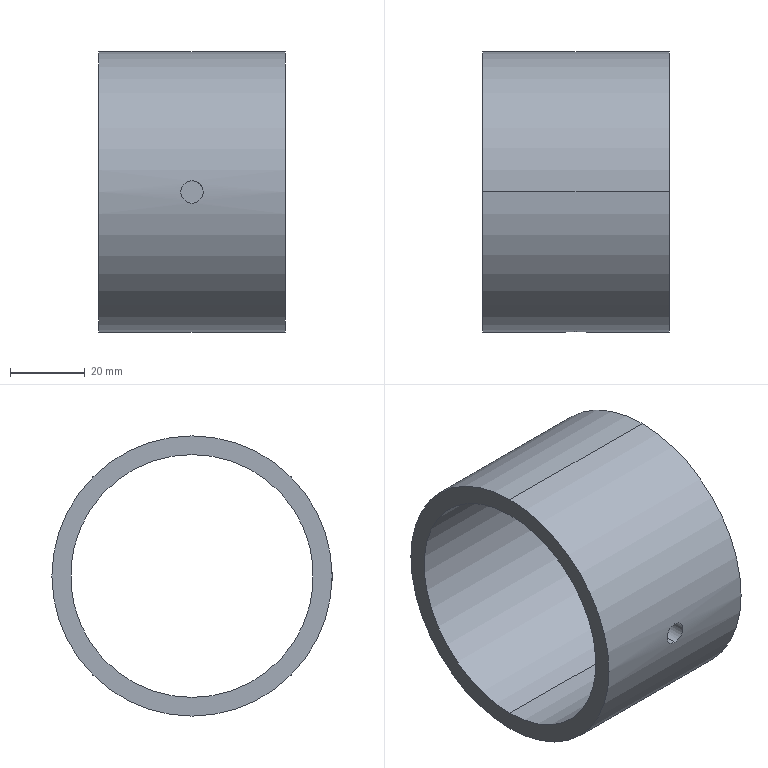Component | SolidWorks | 22Bushing-1 | 1 solid | 8 faces | box 50 x 75 x 75 mm | volume 54836 mm3 | cylinder 6 | plane 2 | commonest cylinder face diameters 6 x2 65 x2 75 x2
build123d program:
from build123d import *

# Parameters (mm, degrees)
SKETCH10_R          = 37.5
SKETCH10_R_2        = 32.5
BOSS_EXTRUDE4_DEPTH = 25
SKETCH12_R          = 3
CUT_EXTRUDE3_DEPTH  = 59.63


with BuildPart() as part:
    # Sketch10 → Boss-Extrude4 (new, symmetric)
    with BuildSketch(Plane(origin=(0, 0, 0), x_dir=(0, 0, -1), z_dir=(1, 0, 0))):
        Circle(SKETCH10_R)
        Circle(SKETCH10_R_2, mode=Mode.SUBTRACT)
    extrude(amount=BOSS_EXTRUDE4_DEPTH, both=True)

    # Sketch12 → Cut-Extrude3 (cut, through all)
    with BuildSketch(Plane(origin=(0, 0, 0), x_dir=(1, 0, 0), z_dir=(0, 1, 0))):
        with Locations(Location((0, 0, 0), (0, 0, 270))):
            Circle(SKETCH12_R)
    extrude(amount=-CUT_EXTRUDE3_DEPTH, mode=Mode.SUBTRACT)


solid = part.part

# Placed as in the assembly
solid = solid.moved(Location((-35.043, 1.776, 250), (0, 0, 0)))
STEP:
#1=CARTESIAN_POINT('',(-1.38,-1.402,9.724));
#2=VERTEX_POINT('',#1);
#3=CARTESIAN_POINT('',(-1.38,-1.402,9.961));
#4=VERTEX_POINT('',#3);
#5=CARTESIAN_POINT('',(-1.38,-1.402,9.724));
#6=CARTESIAN_POINT('',(-1.387,-1.402,9.724));
#7=CARTESIAN_POINT('',(-1.395,-1.402,9.725));
#8=CARTESIAN_POINT('',(-1.41,-1.402,9.728));
#9=CARTESIAN_POINT('',(-1.418,-1.402,9.73));
#10=CARTESIAN_POINT('',(-1.432,-1.403,9.736));
#11=CARTESIAN_POINT('',(-1.439,-1.403,9.74));
#12=CARTESIAN_POINT('',(-1.452,-1.403,9.749));
#13=CARTESIAN_POINT('',(-1.458,-1.404,9.754));
#14=CARTESIAN_POINT('',(-1.469,-1.404,9.764));
#15=CARTESIAN_POINT('',(-1.473,-1.405,9.77));
#16=CARTESIAN_POINT('',(-1.482,-1.405,9.783));
#17=CARTESIAN_POINT('',(-1.486,-1.406,9.79));
#18=CARTESIAN_POINT('',(-1.495,-1.406,9.811));
#19=CARTESIAN_POINT('',(-1.498,-1.406,9.827));
#20=CARTESIAN_POINT('',(-1.498,-1.406,9.85));
#21=CARTESIAN_POINT('',(-1.497,-1.406,9.858));
#22=CARTESIAN_POINT('',(-1.494,-1.406,9.873));
#23=CARTESIAN_POINT('',(-1.492,-1.406,9.881));
#24=CARTESIAN_POINT('',(-1.486,-1.406,9.895));
#25=CARTESIAN_POINT('',(-1.482,-1.405,9.902));
#26=CARTESIAN_POINT('',(-1.474,-1.405,9.915));
#27=CARTESIAN_POINT('',(-1.469,-1.404,9.921));
#28=CARTESIAN_POINT('',(-1.458,-1.404,9.932));
#29=CARTESIAN_POINT('',(-1.452,-1.403,9.936));
#30=CARTESIAN_POINT('',(-1.439,-1.403,9.945));
#31=CARTESIAN_POINT('',(-1.432,-1.403,9.949));
#32=CARTESIAN_POINT('',(-1.418,-1.402,9.955));
#33=CARTESIAN_POINT('',(-1.41,-1.402,9.957));
#34=CARTESIAN_POINT('',(-1.395,-1.402,9.96));
#35=CARTESIAN_POINT('',(-1.387,-1.402,9.961));
#36=CARTESIAN_POINT('',(-1.38,-1.402,9.961));
#37=B_SPLINE_CURVE_WITH_KNOTS('',3,(#5,#6,#7,#8,#9,#10,#11,#12,#13,#14,#15,#16,#17,#18,#19,#20,#21,#22,#23,#24,#25,#26,#27,#28,#29,#30,#31,#32,#33,#34,#35,#36),.UNSPECIFIED.,.F.,.F.,(4,2,2,2,2,2,2,2,2,2,2,2,2,2,2,4),(0.01408,0.01466,0.01525,0.01583,0.01642,0.01701,0.01759,0.01877,0.01935,0.01994,0.02053,0.02111,0.0217,0.02228,0.02287,0.02346),.UNSPECIFIED.);
#38=EDGE_CURVE('',#2,#4,#37,.T.);
#39=ORIENTED_EDGE('',*,*,#38,.F.);
#40=CARTESIAN_POINT('',(-1.38,-1.204,9.724));
#41=VERTEX_POINT('',#40);
#42=CARTESIAN_POINT('',(-1.38,-1.406,9.724));
#43=DIRECTION('',(0.,1.,0.));
#44=VECTOR('',#43,39.37);
#45=LINE('',#42,#44);
#46=EDGE_CURVE('',#2,#41,#45,.T.);
#47=ORIENTED_EDGE('',*,*,#46,.T.);
#48=CARTESIAN_POINT('',(-1.38,-1.204,9.961));
#49=VERTEX_POINT('',#48);
#50=CARTESIAN_POINT('',(-1.38,-1.204,9.724));
#51=CARTESIAN_POINT('',(-1.387,-1.204,9.724));
#52=CARTESIAN_POINT('',(-1.395,-1.204,9.725));
#53=CARTESIAN_POINT('',(-1.41,-1.204,9.728));
#54=CARTESIAN_POINT('',(-1.418,-1.205,9.73));
#55=CARTESIAN_POINT('',(-1.432,-1.205,9.736));
#56=CARTESIAN_POINT('',(-1.439,-1.205,9.74));
#57=CARTESIAN_POINT('',(-1.452,-1.206,9.749));
#58=CARTESIAN_POINT('',(-1.458,-1.207,9.754));
#59=CARTESIAN_POINT('',(-1.469,-1.207,9.764));
#60=CARTESIAN_POINT('',(-1.474,-1.208,9.77));
#61=CARTESIAN_POINT('',(-1.482,-1.208,9.783));
#62=CARTESIAN_POINT('',(-1.486,-1.209,9.79));
#63=CARTESIAN_POINT('',(-1.492,-1.209,9.804));
#64=CARTESIAN_POINT('',(-1.494,-1.209,9.812));
#65=CARTESIAN_POINT('',(-1.497,-1.21,9.827));
#66=CARTESIAN_POINT('',(-1.498,-1.21,9.835));
#67=CARTESIAN_POINT('',(-1.498,-1.21,9.85));
#68=CARTESIAN_POINT('',(-1.497,-1.21,9.858));
#69=CARTESIAN_POINT('',(-1.494,-1.209,9.873));
#70=CARTESIAN_POINT('',(-1.492,-1.209,9.881));
#71=CARTESIAN_POINT('',(-1.486,-1.209,9.895));
#72=CARTESIAN_POINT('',(-1.482,-1.208,9.902));
#73=CARTESIAN_POINT('',(-1.474,-1.208,9.914));
#74=CARTESIAN_POINT('',(-1.469,-1.207,9.921));
#75=CARTESIAN_POINT('',(-1.458,-1.207,9.931));
#76=CARTESIAN_POINT('',(-1.452,-1.206,9.936));
#77=CARTESIAN_POINT('',(-1.439,-1.206,9.945));
#78=CARTESIAN_POINT('',(-1.432,-1.205,9.949));
#79=CARTESIAN_POINT('',(-1.411,-1.204,9.957));
#80=CARTESIAN_POINT('',(-1.395,-1.204,9.961));
#81=CARTESIAN_POINT('',(-1.38,-1.204,9.961));
#82=B_SPLINE_CURVE_WITH_KNOTS('',3,(#50,#51,#52,#53,#54,#55,#56,#57,#58,#59,#60,#61,#62,#63,#64,#65,#66,#67,#68,#69,#70,#71,#72,#73,#74,#75,#76,#77,#78,#79,#80,#81),.UNSPECIFIED.,.F.,.F.,(4,2,2,2,2,2,2,2,2,2,2,2,2,2,2,4),(0.009384,0.009971,0.01056,0.01114,0.01173,0.01232,0.0129,0.01349,0.01408,0.01466,0.01525,0.01583,0.01642,0.01701,0.01759,0.01877),.UNSPECIFIED.);
#83=EDGE_CURVE('',#41,#49,#82,.T.);
#84=ORIENTED_EDGE('',*,*,#83,.T.);
#85=CARTESIAN_POINT('',(-1.38,-1.406,9.961));
#86=DIRECTION('',(0.,1.,0.));
#87=VECTOR('',#86,39.37);
#88=LINE('',#85,#87);
#89=EDGE_CURVE('',#4,#49,#88,.T.);
#90=ORIENTED_EDGE('',*,*,#89,.F.);
#91=EDGE_LOOP('',(#39,#47,#84,#90));
#92=FACE_OUTER_BOUND('',#91,.T.);
#93=CARTESIAN_POINT('',(-1.38,-1.406,9.843));
#94=DIRECTION('',(0.,1.,0.));
#95=DIRECTION('',(0.,0.,1.));
#96=AXIS2_PLACEMENT_3D('',#93,#94,#95);
#97=CYLINDRICAL_SURFACE('',#96,0.1181);
#98=ADVANCED_FACE('',(#92),#97,.F.);
#99=CARTESIAN_POINT('',(-1.38,-1.204,9.961));
#100=CARTESIAN_POINT('',(-1.372,-1.204,9.961));
#101=CARTESIAN_POINT('',(-1.364,-1.204,9.96));
#102=CARTESIAN_POINT('',(-1.349,-1.204,9.957));
#103=CARTESIAN_POINT('',(-1.342,-1.205,9.955));
#104=CARTESIAN_POINT('',(-1.327,-1.205,9.949));
#105=CARTESIAN_POINT('',(-1.32,-1.205,9.945));
#106=CARTESIAN_POINT('',(-1.308,-1.206,9.936));
#107=CARTESIAN_POINT('',(-1.302,-1.207,9.931));
#108=CARTESIAN_POINT('',(-1.291,-1.207,9.921));
#109=CARTESIAN_POINT('',(-1.286,-1.208,9.915));
#110=CARTESIAN_POINT('',(-1.277,-1.208,9.902));
#111=CARTESIAN_POINT('',(-1.273,-1.209,9.895));
#112=CARTESIAN_POINT('',(-1.268,-1.209,9.881));
#113=CARTESIAN_POINT('',(-1.265,-1.209,9.873));
#114=CARTESIAN_POINT('',(-1.262,-1.21,9.858));
#115=CARTESIAN_POINT('',(-1.262,-1.21,9.85));
#116=CARTESIAN_POINT('',(-1.262,-1.21,9.835));
#117=CARTESIAN_POINT('',(-1.262,-1.21,9.827));
#118=CARTESIAN_POINT('',(-1.265,-1.209,9.812));
#119=CARTESIAN_POINT('',(-1.268,-1.209,9.805));
#120=CARTESIAN_POINT('',(-1.273,-1.209,9.79));
#121=CARTESIAN_POINT('',(-1.277,-1.208,9.783));
#122=CARTESIAN_POINT('',(-1.286,-1.208,9.77));
#123=CARTESIAN_POINT('',(-1.291,-1.207,9.765));
#124=CARTESIAN_POINT('',(-1.302,-1.207,9.754));
#125=CARTESIAN_POINT('',(-1.308,-1.206,9.749));
#126=CARTESIAN_POINT('',(-1.32,-1.206,9.74));
#127=CARTESIAN_POINT('',(-1.327,-1.205,9.736));
#128=CARTESIAN_POINT('',(-1.342,-1.205,9.73));
#129=CARTESIAN_POINT('',(-1.349,-1.204,9.728));
#130=CARTESIAN_POINT('',(-1.364,-1.204,9.725));
#131=CARTESIAN_POINT('',(-1.372,-1.204,9.724));
#132=CARTESIAN_POINT('',(-1.38,-1.204,9.724));
#133=B_SPLINE_CURVE_WITH_KNOTS('',3,(#99,#100,#101,#102,#103,#104,#105,#106,#107,#108,#109,#110,#111,#112,#113,#114,#115,#116,#117,#118,#119,#120,#121,#122,#123,#124,#125,#126,#127,#128,#129,#130,#131,#132),.UNSPECIFIED.,.F.,.F.,(4,2,2,2,2,2,2,2,2,2,2,2,2,2,2,2,4),(0.,0.0005865,0.001173,0.00176,0.002346,0.002933,0.003519,0.004106,0.004692,0.005279,0.005865,0.006452,0.007038,0.007625,0.008211,0.008798,0.009384),.UNSPECIFIED.);
#134=EDGE_CURVE('',#49,#41,#133,.T.);
#135=ORIENTED_EDGE('',*,*,#134,.F.);
#136=ORIENTED_EDGE('',*,*,#83,.F.);
#137=EDGE_LOOP('',(#135,#136));
#138=FACE_BOUND('',#137,.T.);
#139=CARTESIAN_POINT('',(-0.3954,0.06992,11.122));
#140=VERTEX_POINT('',#139);
#141=CARTESIAN_POINT('',(-0.3954,0.06992,8.563));
#142=VERTEX_POINT('',#141);
#143=CARTESIAN_POINT('',(-0.3954,0.06992,9.843));
#144=DIRECTION('',(1.,0.,0.));
#145=DIRECTION('',(0.,0.,-1.));
#146=AXIS2_PLACEMENT_3D('',#143,#144,#145);
#147=CIRCLE('',#146,1.28);
#148=EDGE_CURVE('',#140,#142,#147,.T.);
#149=ORIENTED_EDGE('',*,*,#148,.T.);
#150=CARTESIAN_POINT('',(-2.364,0.06992,8.563));
#151=VERTEX_POINT('',#150);
#152=CARTESIAN_POINT('',(-0.3954,0.06992,8.563));
#153=DIRECTION('',(-1.,0.,0.));
#154=VECTOR('',#153,39.37);
#155=LINE('',#152,#154);
#156=EDGE_CURVE('',#142,#151,#155,.T.);
#157=ORIENTED_EDGE('',*,*,#156,.T.);
#158=CARTESIAN_POINT('',(-2.364,0.06992,11.122));
#159=VERTEX_POINT('',#158);
#160=CARTESIAN_POINT('',(-2.364,0.06992,9.843));
#161=DIRECTION('',(1.,0.,0.));
#162=DIRECTION('',(0.,0.,-1.));
#163=AXIS2_PLACEMENT_3D('',#160,#161,#162);
#164=CIRCLE('',#163,1.28);
#165=EDGE_CURVE('',#159,#151,#164,.T.);
#166=ORIENTED_EDGE('',*,*,#165,.F.);
#167=CARTESIAN_POINT('',(-0.3954,0.06992,11.122));
#168=DIRECTION('',(-1.,0.,0.));
#169=VECTOR('',#168,39.37);
#170=LINE('',#167,#169);
#171=EDGE_CURVE('',#140,#159,#170,.T.);
#172=ORIENTED_EDGE('',*,*,#171,.F.);
#173=EDGE_LOOP('',(#149,#157,#166,#172));
#174=FACE_OUTER_BOUND('',#173,.T.);
#175=CARTESIAN_POINT('',(-0.3954,0.06992,9.843));
#176=DIRECTION('',(-1.,0.,0.));
#177=DIRECTION('',(0.,0.,1.));
#178=AXIS2_PLACEMENT_3D('',#175,#176,#177);
#179=CYLINDRICAL_SURFACE('',#178,1.28);
#180=ADVANCED_FACE('',(#138,#174),#179,.F.);
#181=CARTESIAN_POINT('',(-0.3954,0.06992,8.366));
#182=VERTEX_POINT('',#181);
#183=CARTESIAN_POINT('',(-0.3954,0.06992,11.319));
#184=VERTEX_POINT('',#183);
#185=CARTESIAN_POINT('',(-0.3954,0.06992,9.843));
#186=DIRECTION('',(1.,0.,0.));
#187=DIRECTION('',(0.,0.,-1.));
#188=AXIS2_PLACEMENT_3D('',#185,#186,#187);
#189=CIRCLE('',#188,1.476);
#190=EDGE_CURVE('',#182,#184,#189,.T.);
#191=ORIENTED_EDGE('',*,*,#190,.F.);
#192=CARTESIAN_POINT('',(-2.364,0.06992,8.366));
#193=VERTEX_POINT('',#192);
#194=CARTESIAN_POINT('',(-0.3954,0.06992,8.366));
#195=DIRECTION('',(-1.,0.,0.));
#196=VECTOR('',#195,39.37);
#197=LINE('',#194,#196);
#198=EDGE_CURVE('',#182,#193,#197,.T.);
#199=ORIENTED_EDGE('',*,*,#198,.T.);
#200=CARTESIAN_POINT('',(-2.364,0.06992,11.319));
#201=VERTEX_POINT('',#200);
#202=CARTESIAN_POINT('',(-2.364,0.06992,9.843));
#203=DIRECTION('',(1.,0.,0.));
#204=DIRECTION('',(0.,0.,-1.));
#205=AXIS2_PLACEMENT_3D('',#202,#203,#204);
#206=CIRCLE('',#205,1.476);
#207=EDGE_CURVE('',#193,#201,#206,.T.);
#208=ORIENTED_EDGE('',*,*,#207,.T.);
#209=CARTESIAN_POINT('',(-0.3954,0.06992,11.319));
#210=DIRECTION('',(-1.,0.,0.));
#211=VECTOR('',#210,39.37);
#212=LINE('',#209,#211);
#213=EDGE_CURVE('',#184,#201,#212,.T.);
#214=ORIENTED_EDGE('',*,*,#213,.F.);
#215=EDGE_LOOP('',(#191,#199,#208,#214));
#216=FACE_OUTER_BOUND('',#215,.T.);
#217=CARTESIAN_POINT('',(-0.3954,0.06992,9.843));
#218=DIRECTION('',(-1.,0.,0.));
#219=DIRECTION('',(0.,0.,1.));
#220=AXIS2_PLACEMENT_3D('',#217,#218,#219);
#221=CYLINDRICAL_SURFACE('',#220,1.476);
#222=ADVANCED_FACE('',(#216),#221,.T.);
#223=CARTESIAN_POINT('',(-0.3954,0.06992,9.843));
#224=DIRECTION('',(1.,0.,0.));
#225=DIRECTION('',(0.,0.,-1.));
#226=AXIS2_PLACEMENT_3D('',#223,#224,#225);
#227=CIRCLE('',#226,1.476);
#228=EDGE_CURVE('',#184,#182,#227,.T.);
#229=ORIENTED_EDGE('',*,*,#228,.T.);
#230=ORIENTED_EDGE('',*,*,#190,.T.);
#231=EDGE_LOOP('',(#229,#230));
#232=FACE_OUTER_BOUND('',#231,.T.);
#233=ORIENTED_EDGE('',*,*,#148,.F.);
#234=CARTESIAN_POINT('',(-0.3954,0.06992,9.843));
#235=DIRECTION('',(1.,0.,0.));
#236=DIRECTION('',(0.,0.,-1.));
#237=AXIS2_PLACEMENT_3D('',#234,#235,#236);
#238=CIRCLE('',#237,1.28);
#239=EDGE_CURVE('',#142,#140,#238,.T.);
#240=ORIENTED_EDGE('',*,*,#239,.F.);
#241=EDGE_LOOP('',(#233,#240));
#242=FACE_BOUND('',#241,.T.);
#243=CARTESIAN_POINT('',(-0.3954,0.06992,9.843));
#244=DIRECTION('',(1.,0.,0.));
#245=DIRECTION('',(0.,0.,-1.));
#246=AXIS2_PLACEMENT_3D('',#243,#244,#245);
#247=PLANE('',#246);
#248=ADVANCED_FACE('',(#232,#242),#247,.T.);
#249=CARTESIAN_POINT('',(-2.364,0.06992,9.843));
#250=DIRECTION('',(1.,0.,0.));
#251=DIRECTION('',(0.,0.,-1.));
#252=AXIS2_PLACEMENT_3D('',#249,#250,#251);
#253=CIRCLE('',#252,1.476);
#254=EDGE_CURVE('',#201,#193,#253,.T.);
#255=ORIENTED_EDGE('',*,*,#254,.F.);
#256=ORIENTED_EDGE('',*,*,#207,.F.);
#257=EDGE_LOOP('',(#255,#256));
#258=FACE_OUTER_BOUND('',#257,.T.);
#259=ORIENTED_EDGE('',*,*,#165,.T.);
#260=CARTESIAN_POINT('',(-2.364,0.06992,9.843));
#261=DIRECTION('',(1.,0.,0.));
#262=DIRECTION('',(0.,0.,-1.));
#263=AXIS2_PLACEMENT_3D('',#260,#261,#262);
#264=CIRCLE('',#263,1.28);
#265=EDGE_CURVE('',#151,#159,#264,.T.);
#266=ORIENTED_EDGE('',*,*,#265,.T.);
#267=EDGE_LOOP('',(#259,#266));
#268=FACE_BOUND('',#267,.T.);
#269=CARTESIAN_POINT('',(-2.364,0.06992,9.843));
#270=DIRECTION('',(1.,0.,0.));
#271=DIRECTION('',(0.,0.,-1.));
#272=AXIS2_PLACEMENT_3D('',#269,#270,#271);
#273=PLANE('',#272);
#274=ADVANCED_FACE('',(#258,#268),#273,.F.);
#275=ORIENTED_EDGE('',*,*,#198,.F.);
#276=ORIENTED_EDGE('',*,*,#228,.F.);
#277=ORIENTED_EDGE('',*,*,#213,.T.);
#278=ORIENTED_EDGE('',*,*,#254,.T.);
#279=EDGE_LOOP('',(#275,#276,#277,#278));
#280=FACE_OUTER_BOUND('',#279,.T.);
#281=CARTESIAN_POINT('',(-1.38,-1.402,9.961));
#282=CARTESIAN_POINT('',(-1.372,-1.402,9.961));
#283=CARTESIAN_POINT('',(-1.364,-1.402,9.96));
#284=CARTESIAN_POINT('',(-1.349,-1.402,9.957));
#285=CARTESIAN_POINT('',(-1.342,-1.402,9.955));
#286=CARTESIAN_POINT('',(-1.327,-1.403,9.949));
#287=CARTESIAN_POINT('',(-1.32,-1.403,9.945));
#288=CARTESIAN_POINT('',(-1.308,-1.403,9.936));
#289=CARTESIAN_POINT('',(-1.302,-1.404,9.932));
#290=CARTESIAN_POINT('',(-1.291,-1.404,9.921));
#291=CARTESIAN_POINT('',(-1.286,-1.405,9.915));
#292=CARTESIAN_POINT('',(-1.277,-1.405,9.902));
#293=CARTESIAN_POINT('',(-1.273,-1.406,9.895));
#294=CARTESIAN_POINT('',(-1.268,-1.406,9.881));
#295=CARTESIAN_POINT('',(-1.265,-1.406,9.873));
#296=CARTESIAN_POINT('',(-1.262,-1.406,9.858));
#297=CARTESIAN_POINT('',(-1.262,-1.406,9.85));
#298=CARTESIAN_POINT('',(-1.262,-1.406,9.835));
#299=CARTESIAN_POINT('',(-1.262,-1.406,9.827));
#300=CARTESIAN_POINT('',(-1.265,-1.406,9.812));
#301=CARTESIAN_POINT('',(-1.268,-1.406,9.804));
#302=CARTESIAN_POINT('',(-1.273,-1.406,9.79));
#303=CARTESIAN_POINT('',(-1.277,-1.405,9.783));
#304=CARTESIAN_POINT('',(-1.286,-1.405,9.77));
#305=CARTESIAN_POINT('',(-1.291,-1.404,9.764));
#306=CARTESIAN_POINT('',(-1.302,-1.404,9.754));
#307=CARTESIAN_POINT('',(-1.308,-1.403,9.749));
#308=CARTESIAN_POINT('',(-1.32,-1.403,9.74));
#309=CARTESIAN_POINT('',(-1.327,-1.403,9.736));
#310=CARTESIAN_POINT('',(-1.342,-1.402,9.73));
#311=CARTESIAN_POINT('',(-1.349,-1.402,9.728));
#312=CARTESIAN_POINT('',(-1.364,-1.402,9.725));
#313=CARTESIAN_POINT('',(-1.372,-1.402,9.724));
#314=CARTESIAN_POINT('',(-1.38,-1.402,9.724));
#315=B_SPLINE_CURVE_WITH_KNOTS('',3,(#281,#282,#283,#284,#285,#286,#287,#288,#289,#290,#291,#292,#293,#294,#295,#296,#297,#298,#299,#300,#301,#302,#303,#304,#305,#306,#307,#308,#309,#310,#311,#312,#313,#314),.UNSPECIFIED.,.F.,.F.,(4,2,2,2,2,2,2,2,2,2,2,2,2,2,2,2,4),(0.004693,0.005279,0.005866,0.006452,0.007038,0.007625,0.008211,0.008798,0.009384,0.009971,0.01056,0.01114,0.01173,0.01232,0.0129,0.01349,0.01408),.UNSPECIFIED.);
#316=EDGE_CURVE('',#4,#2,#315,.T.);
#317=ORIENTED_EDGE('',*,*,#316,.T.);
#318=ORIENTED_EDGE('',*,*,#38,.T.);
#319=EDGE_LOOP('',(#317,#318));
#320=FACE_BOUND('',#319,.T.);
#321=CARTESIAN_POINT('',(-0.3954,0.06992,9.843));
#322=DIRECTION('',(-1.,0.,0.));
#323=DIRECTION('',(0.,0.,1.));
#324=AXIS2_PLACEMENT_3D('',#321,#322,#323);
#325=CYLINDRICAL_SURFACE('',#324,1.476);
#326=ADVANCED_FACE('',(#280,#320),#325,.T.);
#327=ORIENTED_EDGE('',*,*,#156,.F.);
#328=ORIENTED_EDGE('',*,*,#239,.T.);
#329=ORIENTED_EDGE('',*,*,#171,.T.);
#330=ORIENTED_EDGE('',*,*,#265,.F.);
#331=EDGE_LOOP('',(#327,#328,#329,#330));
#332=FACE_OUTER_BOUND('',#331,.T.);
#333=CARTESIAN_POINT('',(-0.3954,0.06992,9.843));
#334=DIRECTION('',(-1.,0.,0.));
#335=DIRECTION('',(0.,0.,1.));
#336=AXIS2_PLACEMENT_3D('',#333,#334,#335);
#337=CYLINDRICAL_SURFACE('',#336,1.28);
#338=ADVANCED_FACE('',(#332),#337,.F.);
#339=ORIENTED_EDGE('',*,*,#46,.F.);
#340=ORIENTED_EDGE('',*,*,#316,.F.);
#341=ORIENTED_EDGE('',*,*,#89,.T.);
#342=ORIENTED_EDGE('',*,*,#134,.T.);
#343=EDGE_LOOP('',(#339,#340,#341,#342));
#344=FACE_OUTER_BOUND('',#343,.T.);
#345=CARTESIAN_POINT('',(-1.38,-1.406,9.843));
#346=DIRECTION('',(0.,1.,0.));
#347=DIRECTION('',(0.,0.,1.));
#348=AXIS2_PLACEMENT_3D('',#345,#346,#347);
#349=CYLINDRICAL_SURFACE('',#348,0.1181);
#350=ADVANCED_FACE('',(#344),#349,.F.);
#351=CLOSED_SHELL('',(#98,#180,#222,#248,#274,#326,#338,#350));
#352=MANIFOLD_SOLID_BREP('',#351);
#353=CARTESIAN_POINT('',(0.,0.,0.));
#354=DIRECTION('',(0.,0.,1.));
#355=DIRECTION('',(1.,0.,0.));
#356=AXIS2_PLACEMENT_3D('',#353,#354,#355);
#357=(LENGTH_UNIT()NAMED_UNIT(*)SI_UNIT($,.METRE.));
#358=LENGTH_MEASURE_WITH_UNIT(LENGTH_MEASURE(0.0254),#357);
#359=DIMENSIONAL_EXPONENTS(1.,0.,0.,0.,0.,0.,0.);
#360=(CONVERSION_BASED_UNIT('',#358)LENGTH_UNIT()NAMED_UNIT(#359));
#361=UNCERTAINTY_MEASURE_WITH_UNIT(LENGTH_MEASURE(0.00001),#360,'','');
#362=(NAMED_UNIT(*)PLANE_ANGLE_UNIT()SI_UNIT($,.RADIAN.));
#363=(NAMED_UNIT(*)SI_UNIT($,.STERADIAN.)SOLID_ANGLE_UNIT());
#364=(GEOMETRIC_REPRESENTATION_CONTEXT(3)GLOBAL_UNCERTAINTY_ASSIGNED_CONTEXT((#361))GLOBAL_UNIT_ASSIGNED_CONTEXT((#360,#362,#363))REPRESENTATION_CONTEXT('',''));
#365=ADVANCED_BREP_SHAPE_REPRESENTATION('',(#352,#356),#364);
#366=COLOUR_RGB('',0.7922,0.8196,0.9333);
#367=FILL_AREA_STYLE_COLOUR('',#366);
#368=FILL_AREA_STYLE('',(#367));
#369=SURFACE_STYLE_FILL_AREA(#368);
#370=SURFACE_SIDE_STYLE('',(#369));
#371=SURFACE_STYLE_USAGE(.BOTH.,#370);
#372=PRESENTATION_STYLE_ASSIGNMENT((#371));
#373=STYLED_ITEM('',(#372),#352);
#374=(LENGTH_UNIT()NAMED_UNIT(*)SI_UNIT($,.METRE.));
#375=LENGTH_MEASURE_WITH_UNIT(LENGTH_MEASURE(0.0254),#374);
#376=DIMENSIONAL_EXPONENTS(1.,0.,0.,0.,0.,0.,0.);
#377=(CONVERSION_BASED_UNIT('',#375)LENGTH_UNIT()NAMED_UNIT(#376));
#378=UNCERTAINTY_MEASURE_WITH_UNIT(LENGTH_MEASURE(0.00001),#377,'','');
#379=(NAMED_UNIT(*)PLANE_ANGLE_UNIT()SI_UNIT($,.RADIAN.));
#380=(NAMED_UNIT(*)SI_UNIT($,.STERADIAN.)SOLID_ANGLE_UNIT());
#381=(GEOMETRIC_REPRESENTATION_CONTEXT(3)GLOBAL_UNCERTAINTY_ASSIGNED_CONTEXT((#378))GLOBAL_UNIT_ASSIGNED_CONTEXT((#377,#379,#380))REPRESENTATION_CONTEXT('',''));
#382=MECHANICAL_DESIGN_GEOMETRIC_PRESENTATION_REPRESENTATION('',(#373),#381);
#383=PRESENTATION_LAYER_ASSIGNMENT('','',(#373));